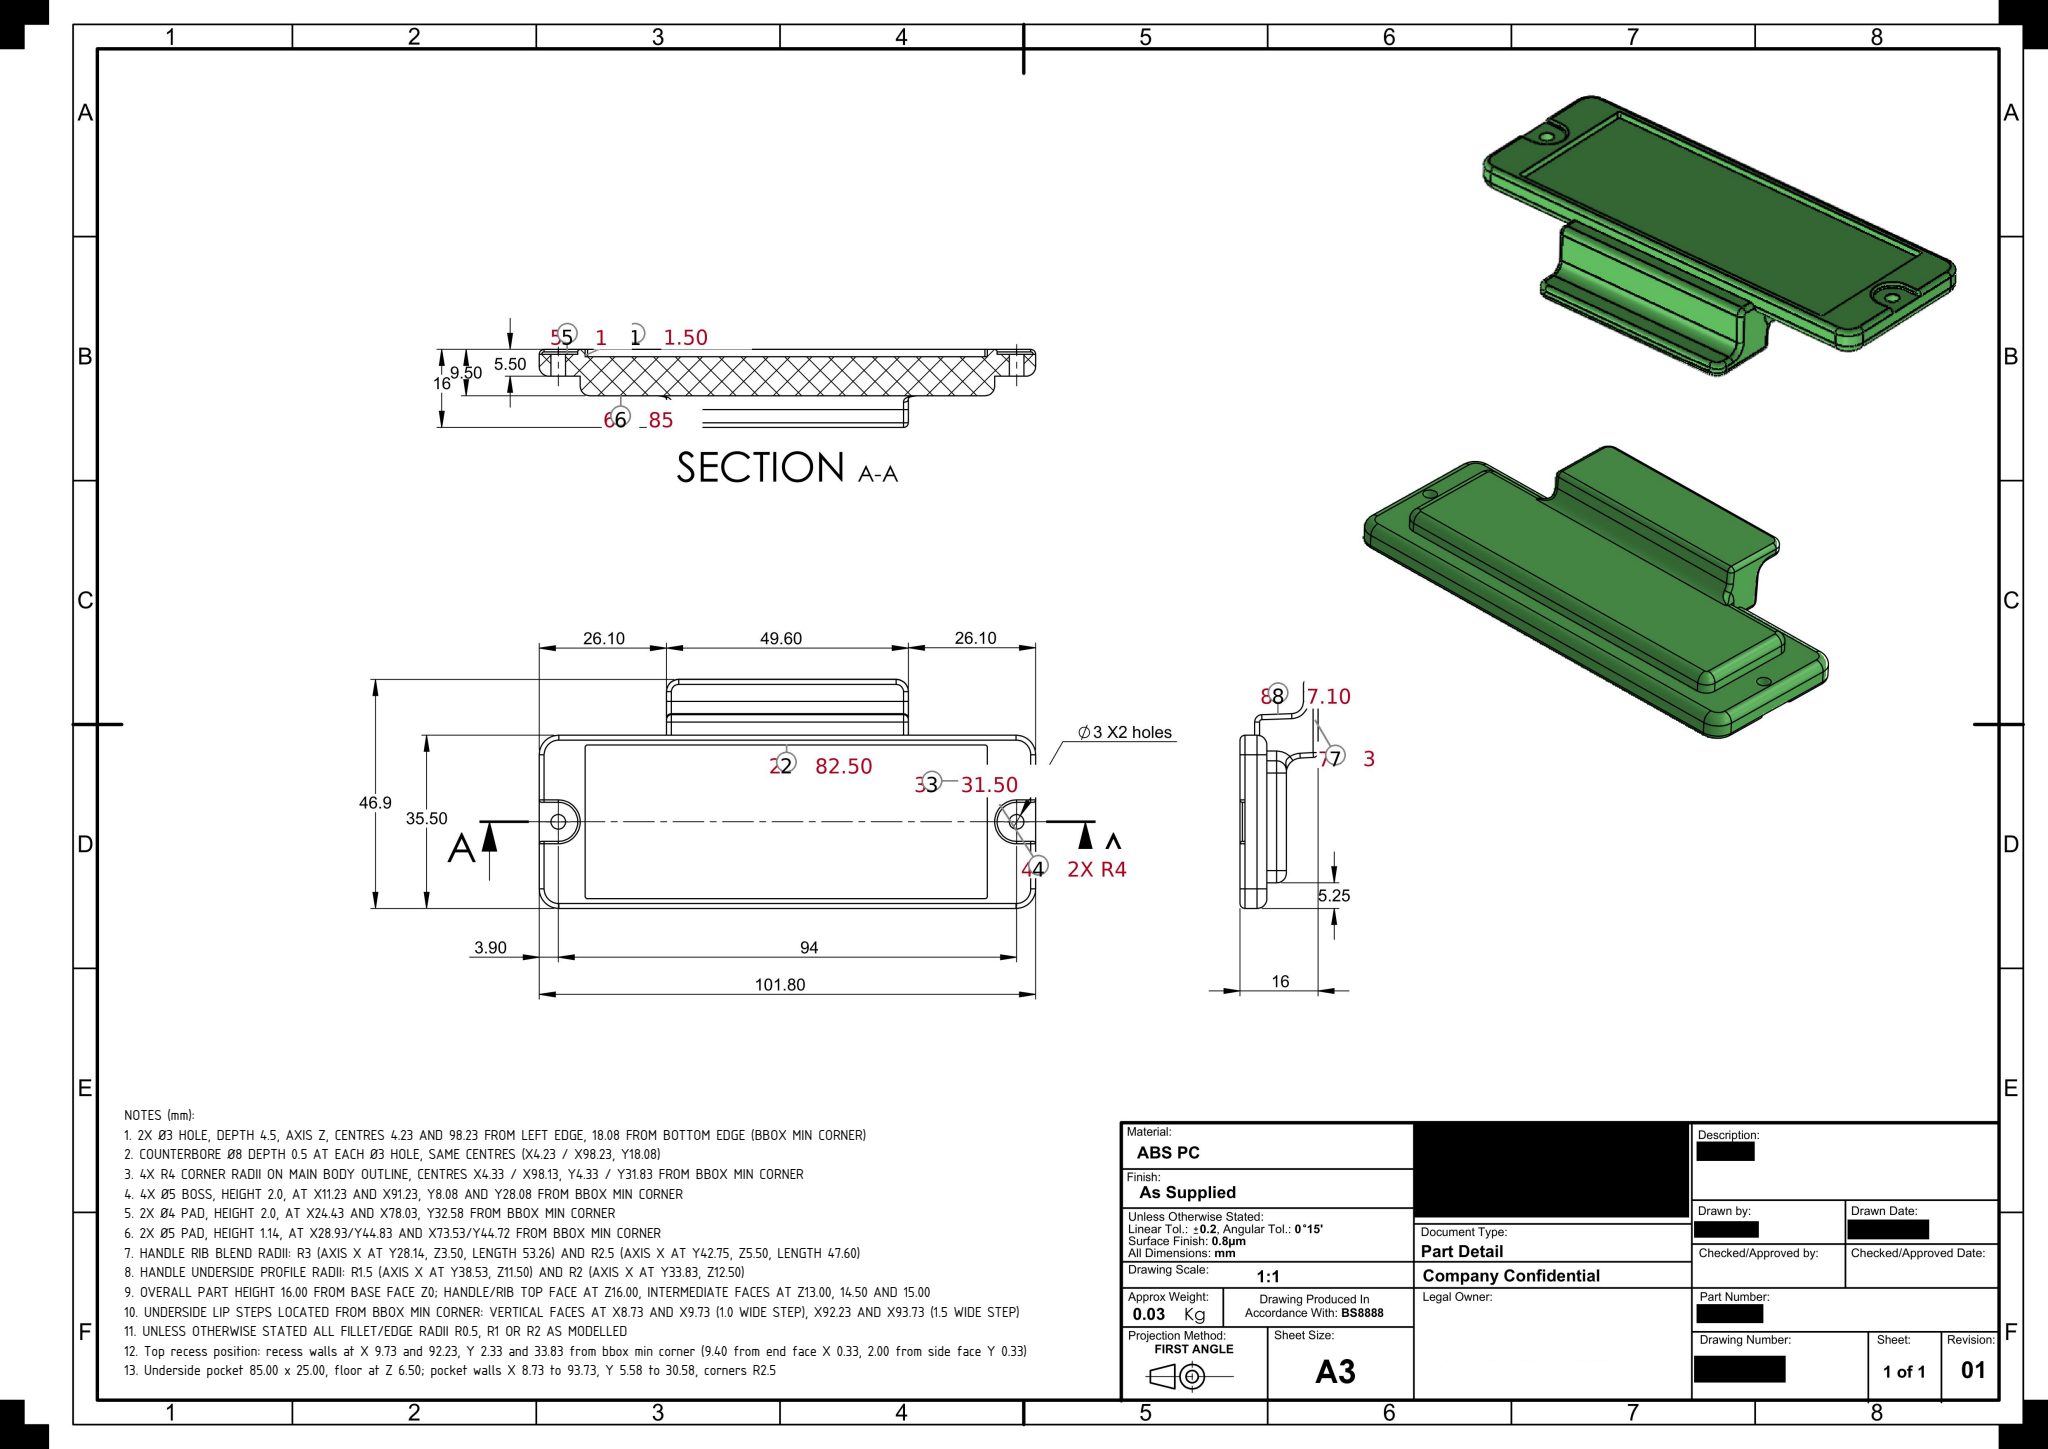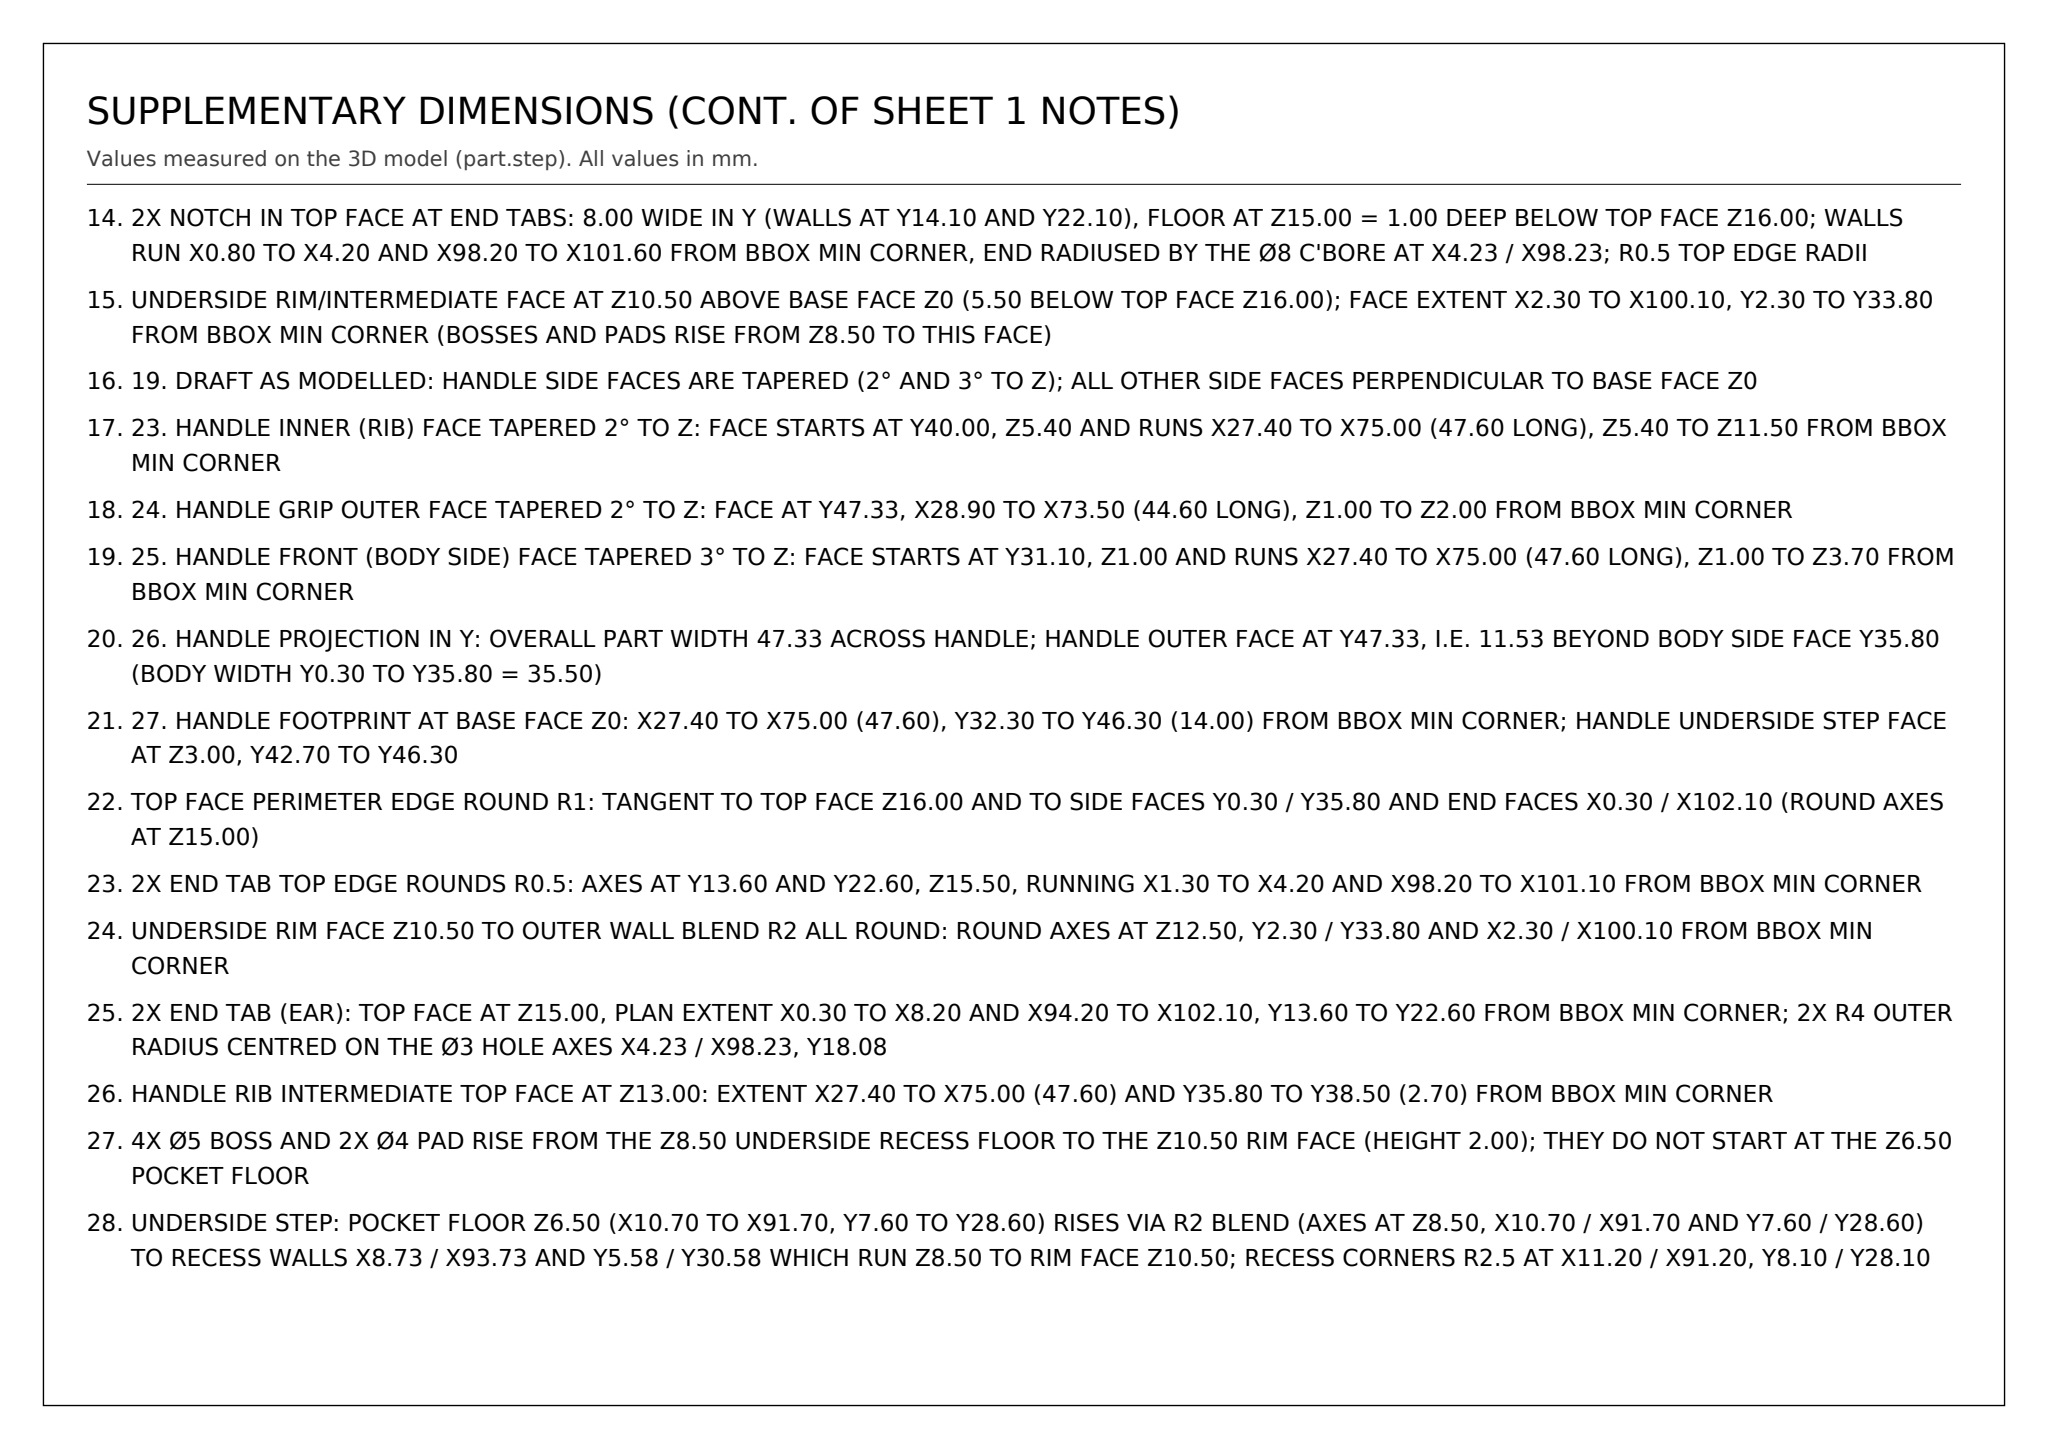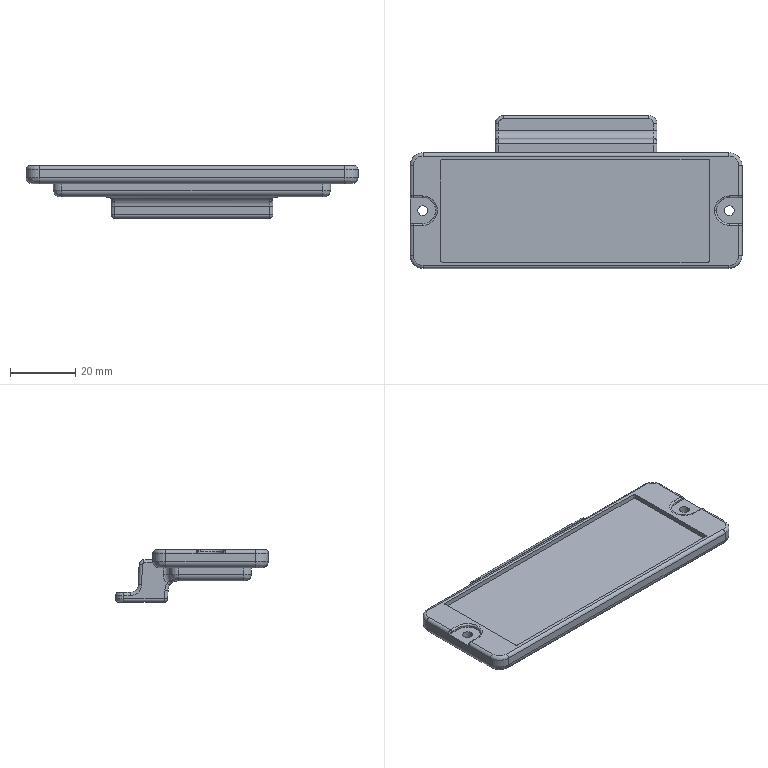Part | SolidWorks | mm | material ABS PC | 1 solid | 128 faces | box 101.8 x 46.96 x 16 mm | volume 30298 mm3 | cylinder 61 | plane 32 | spline 19 | torus 14 | sphere 2 | commonest cylinder face diameters 2 x20 4 x13 1 x8 8 x7 5 x7 3 x5 6 x1
Drawing notes:
2X Ø3 HOLE, DEPTH 4.5, AXIS Z, CENTRES 4.23 AND 98.23 FROM LEFT EDGE, 18.08 FROM BOTTOM EDGE (BBOX MIN CORNER) | from the solid: cylinders[3.0,'z',[4.23,18.08],4.5] and [3.0,'z',[98.23,18.08],4.5]
COUNTERBORE Ø8 DEPTH 0.5 AT EACH Ø3 HOLE, SAME CENTRES (X4.23 / X98.23, Y18.08) | from the solid: cylinders[8.0,'z',[4.23,18.08],0.5] and [8.0,'z',[98.23,18.08],0.5]
4X R4 CORNER RADII ON MAIN BODY OUTLINE, CENTRES X4.33 / X98.13, Y4.33 / Y31.83 FROM BBOX MIN CORNER | from the solid: cylinders[8.0,'z',[4.33,4.33],2.5], [8.0,'z',[4.33,31.83],2.5], [8.0,'z',[98.13,4.33],2.5], [8.0,'z',[98.13,31.83],2.5]
4X Ø5 BOSS, HEIGHT 2.0, AT X11.23 AND X91.23, Y8.08 AND Y28.08 FROM BBOX MIN CORNER | from the solid: cylinders[5.0,'z',[11.23,8.08],2.0], [5.0,'z',[11.23,28.08],2.0], [5.0,'z',[91.23,8.08],2.0], [5.0,'z',[91.23,28.08],2.0]
2X Ø4 PAD, HEIGHT 2.0, AT X24.43 AND X78.03, Y32.58 FROM BBOX MIN CORNER | from the solid: cylinders[4.0,'z',[24.43,32.58],2.0] and [4.0,'z',[78.03,32.58],2.0]
2X Ø5 PAD, HEIGHT 1.14, AT X28.93/Y44.83 AND X73.53/Y44.72 FROM BBOX MIN CORNER | from the solid: cylinders[5.0,'z',[28.93,44.83],1.14] and [5.0,'z',[73.53,44.72],1.14]
HANDLE RIB BLEND RADII: R3 (AXIS X AT Y28.14, Z3.50, LENGTH 53.26) AND R2.5 (AXIS X AT Y42.75, Z5.50, LENGTH 47.60) | from the solid: cylinders[6.0,'x',[null,28.14,3.5],53.26] and [5.0,'x',[null,42.75,5.5],47.6]
HANDLE UNDERSIDE PROFILE RADII: R1.5 (AXIS X AT Y38.53, Z11.50) AND R2 (AXIS X AT Y33.83, Z12.50) | from the solid: cylinders[3.0,'x',[null,38.53,11.5],47.6] and [4.0,'x',[null,33.83,12.5],22.23]
OVERALL PART HEIGHT 16.00 FROM BASE FACE Z0; HANDLE/RIB TOP FACE AT Z16.00, INTERMEDIATE FACES AT Z13.00, 14.50 AND 15.00 | from the solid: axis_planes z offsets 0.0, 13.0, 14.5, 15.0, 16.0
UNDERSIDE LIP STEPS LOCATED FROM BBOX MIN CORNER: VERTICAL FACES AT X8.73 AND X9.73 (1.0 WIDE STEP), X92.23 AND X93.73 (1.5 WIDE STEP) | from the solid: axis_planes x offsets 8.73, 9.73, 92.23, 93.73
UNLESS OTHERWISE STATED ALL FILLET/EDGE RADII R0.5, R1 OR R2 AS MODELLED | from the solid: fillet_radii [[0.5,3],[1.0,8],[2.0,3]]
Top recess position: recess walls at X 9.73 and 92.23, Y 2.33 and 33.83 from bbox min corner (9.40 from end face X 0.33, 2.00 from side face Y 0.33) | from the solid: axis_planes x 9.73, x 92.23, y 2.33, y 33.83, x 0.33, y 0.33
Underside pocket 85.00 x 25.00, floor at Z 6.50; pocket walls X 8.73 to 93.73, Y 5.58 to 30.58, corners R2.5 | from the solid: cylinders [5.0,'z',[11.23,8.08],2.0] x4 (R2.5); axis_planes x 8.73, x 93.73, y 5.58, y 30.58, z 6.5
2X NOTCH IN TOP FACE AT END TABS: 8.00 WIDE IN Y (WALLS AT Y14.10 AND Y22.10), FLOOR AT Z15.00 = 1.00 DEEP BELOW TOP FACE Z16.00; WALLS RUN X0.80 TO X4.20 AND X98.20 TO X101.60 FROM BBOX MIN CORNER, END RADIUSED BY THE Ø8 C'BORE AT X4.23 / X98.23; R0.5 TOP EDGE RADII | from the solid: axis_planes z offset 15.0 extents x[0.3,8.2] & x[94.2,102.1], y[13.6,22.6]; axis_planes y offset 14.1 and 22.1, x[0.8,4.2] & x[98.2,101.6], z[15.0,15.5]; convex arcs dia 1.0 axis x at (y13.6/y22.6, z15.5); hole/bore dia 8.0 axis z at (4.2,18.1) and (98.2,18.1)
UNDERSIDE RIM/INTERMEDIATE FACE AT Z10.50 ABOVE BASE FACE Z0 (5.50 BELOW TOP FACE Z16.00); FACE EXTENT X2.30 TO X100.10, Y2.30 TO Y33.80 FROM BBOX MIN CORNER (BOSSES AND PADS RISE FROM Z8.50 TO THIS FACE) | from the solid: axis_planes z offset 10.5, extent x[2.3,100.1], y[2.3,33.8], area 781; boss/pad arcs dia 5.0 and 4.0 axis z from 8.5 to 10.5
19. DRAFT AS MODELLED: HANDLE SIDE FACES ARE TAPERED (2° AND 3° TO Z); ALL OTHER SIDE FACES PERPENDICULAR TO BASE FACE Z0 | from the solid: inclined_planes: three faces with angle_to_xyz_axes [90,2,88] and [90,3,87]; all other planes are axis_planes normal to x, y or z
23. HANDLE INNER (RIB) FACE TAPERED 2° TO Z: FACE STARTS AT Y40.00, Z5.40 AND RUNS X27.40 TO X75.00 (47.60 LONG), Z5.40 TO Z11.50 FROM BBOX MIN CORNER | from the solid: inclined_planes: angle [90.0,2.0,88.0], bbox_from [27.4,40.0,5.4], size [47.6,0.2,6.1]
24. HANDLE GRIP OUTER FACE TAPERED 2° TO Z: FACE AT Y47.33, X28.90 TO X73.50 (44.60 LONG), Z1.00 TO Z2.00 FROM BBOX MIN CORNER | from the solid: inclined_planes: angle [90.0,2.0,88.0], bbox_from [28.9,47.3,1.0], size [44.6,0.0,1.0]
25. HANDLE FRONT (BODY SIDE) FACE TAPERED 3° TO Z: FACE STARTS AT Y31.10, Z1.00 AND RUNS X27.40 TO X75.00 (47.60 LONG), Z1.00 TO Z3.70 FROM BBOX MIN CORNER | from the solid: inclined_planes: angle [90.0,3.0,87.0], bbox_from [27.4,31.1,1.0], size [47.6,0.1,2.7]
26. HANDLE PROJECTION IN Y: OVERALL PART WIDTH 47.33 ACROSS HANDLE; HANDLE OUTER FACE AT Y47.33, I.E. 11.53 BEYOND BODY SIDE FACE Y35.80 (BODY WIDTH Y0.30 TO Y35.80 = 35.50) | from the solid: bbox_xyz y=47.335; axis_plane y=35.8 (body side, x4.3-98.1) and y=0.3; inclined plane at y47.3
27. HANDLE FOOTPRINT AT BASE FACE Z0: X27.40 TO X75.00 (47.60), Y32.30 TO Y46.30 (14.00) FROM BBOX MIN CORNER; HANDLE UNDERSIDE STEP FACE AT Z3.00, Y42.70 TO Y46.30 | from the solid: axis_planes z=0.0 extent x[27.4,75.0] y[32.3,46.3]; z=3.0 extent x[27.4,75.0] y[42.7,46.3]
TOP FACE PERIMETER EDGE ROUND R1: TANGENT TO TOP FACE Z16.00 AND TO SIDE FACES Y0.30 / Y35.80 AND END FACES X0.30 / X102.10 (ROUND AXES AT Z15.00) | from the solid: convex arc dia 2.0 axis x at y1.3 and y34.8, z15.0, x4.3-98.1; convex arc dia 2.0 axis y at x1.3 and x101.1, z15.0
2X END TAB TOP EDGE ROUNDS R0.5: AXES AT Y13.60 AND Y22.60, Z15.50, RUNNING X1.30 TO X4.20 AND X98.20 TO X101.10 FROM BBOX MIN CORNER | from the solid: convex arc (round/outer radius) dia 1.0, axis x at [y13.6, z15.5] from x1.3 to 4.2 and from x98.2 to 101.1; convex arc dia 1.0, axis x at [y22.6, z15.5] from x1.3 to 4.2 and from x98.2 to 101.1
UNDERSIDE RIM FACE Z10.50 TO OUTER WALL BLEND R2 ALL ROUND: ROUND AXES AT Z12.50, Y2.30 / Y33.80 AND X2.30 / X100.10 FROM BBOX MIN CORNER | from the solid: convex arc dia 4.0 axis x at y2.3 and y33.8, z12.5; convex arc dia 4.0 axis y at x2.3 and x100.1, z12.5
2X END TAB (EAR): TOP FACE AT Z15.00, PLAN EXTENT X0.30 TO X8.20 AND X94.20 TO X102.10, Y13.60 TO Y22.60 FROM BBOX MIN CORNER; 2X R4 OUTER RADIUS CENTRED ON THE Ø3 HOLE AXES X4.23 / X98.23, Y18.08 | from the solid: axis plane z=15.0 extents x0.3-8.2 and x94.2-102.1, y13.6-22.6; hole/bore dia 3.0 axis z at (4.2,18.1) and (98.2,18.1)
HANDLE RIB INTERMEDIATE TOP FACE AT Z13.00: EXTENT X27.40 TO X75.00 (47.60) AND Y35.80 TO Y38.50 (2.70) FROM BBOX MIN CORNER | from the solid: axis plane z=13.0, extent x 27.4-75.0, y 35.8-38.5
4X Ø5 BOSS AND 2X Ø4 PAD RISE FROM THE Z8.50 UNDERSIDE RECESS FLOOR TO THE Z10.50 RIM FACE (HEIGHT 2.00); THEY DO NOT START AT THE Z6.50 POCKET FLOOR | from the solid: convex arc dia 5.0 axis z at (11.2,8.1),(11.2,28.1),(91.2,8.1),(91.2,28.1) from z8.5 to 10.5; concave arc dia 4.0 axis z at (24.4,32.6) and (78.0,32.6) from z8.5 to 10.5; axis plane z=10.5
UNDERSIDE STEP: POCKET FLOOR Z6.50 (X10.70 TO X91.70, Y7.60 TO Y28.60) RISES VIA R2 BLEND (AXES AT Z8.50, X10.70 / X91.70 AND Y7.60 / Y28.60) TO RECESS WALLS X8.73 / X93.73 AND Y5.58 / Y30.58 WHICH RUN Z8.50 TO RIM FACE Z10.50; RECESS CORNERS R2.5 AT X11.20 / X91.20, Y8.10 / Y28.10 | from the solid: axis plane z=6.5 extent x10.7-91.7, y7.6-28.6; axis planes x8.7 and x93.7 (y8.1-28.1, z8.5-10.5), y5.6 and y30.6 (z8.5-10.5); convex arcs dia 4.0 axis x at y7.6/y28.6 z8.5 and axis y at x10.7/x91.7 z8.5; convex arcs dia 5.0 axis z at (11.2,8.1) etc z8.5-10.5